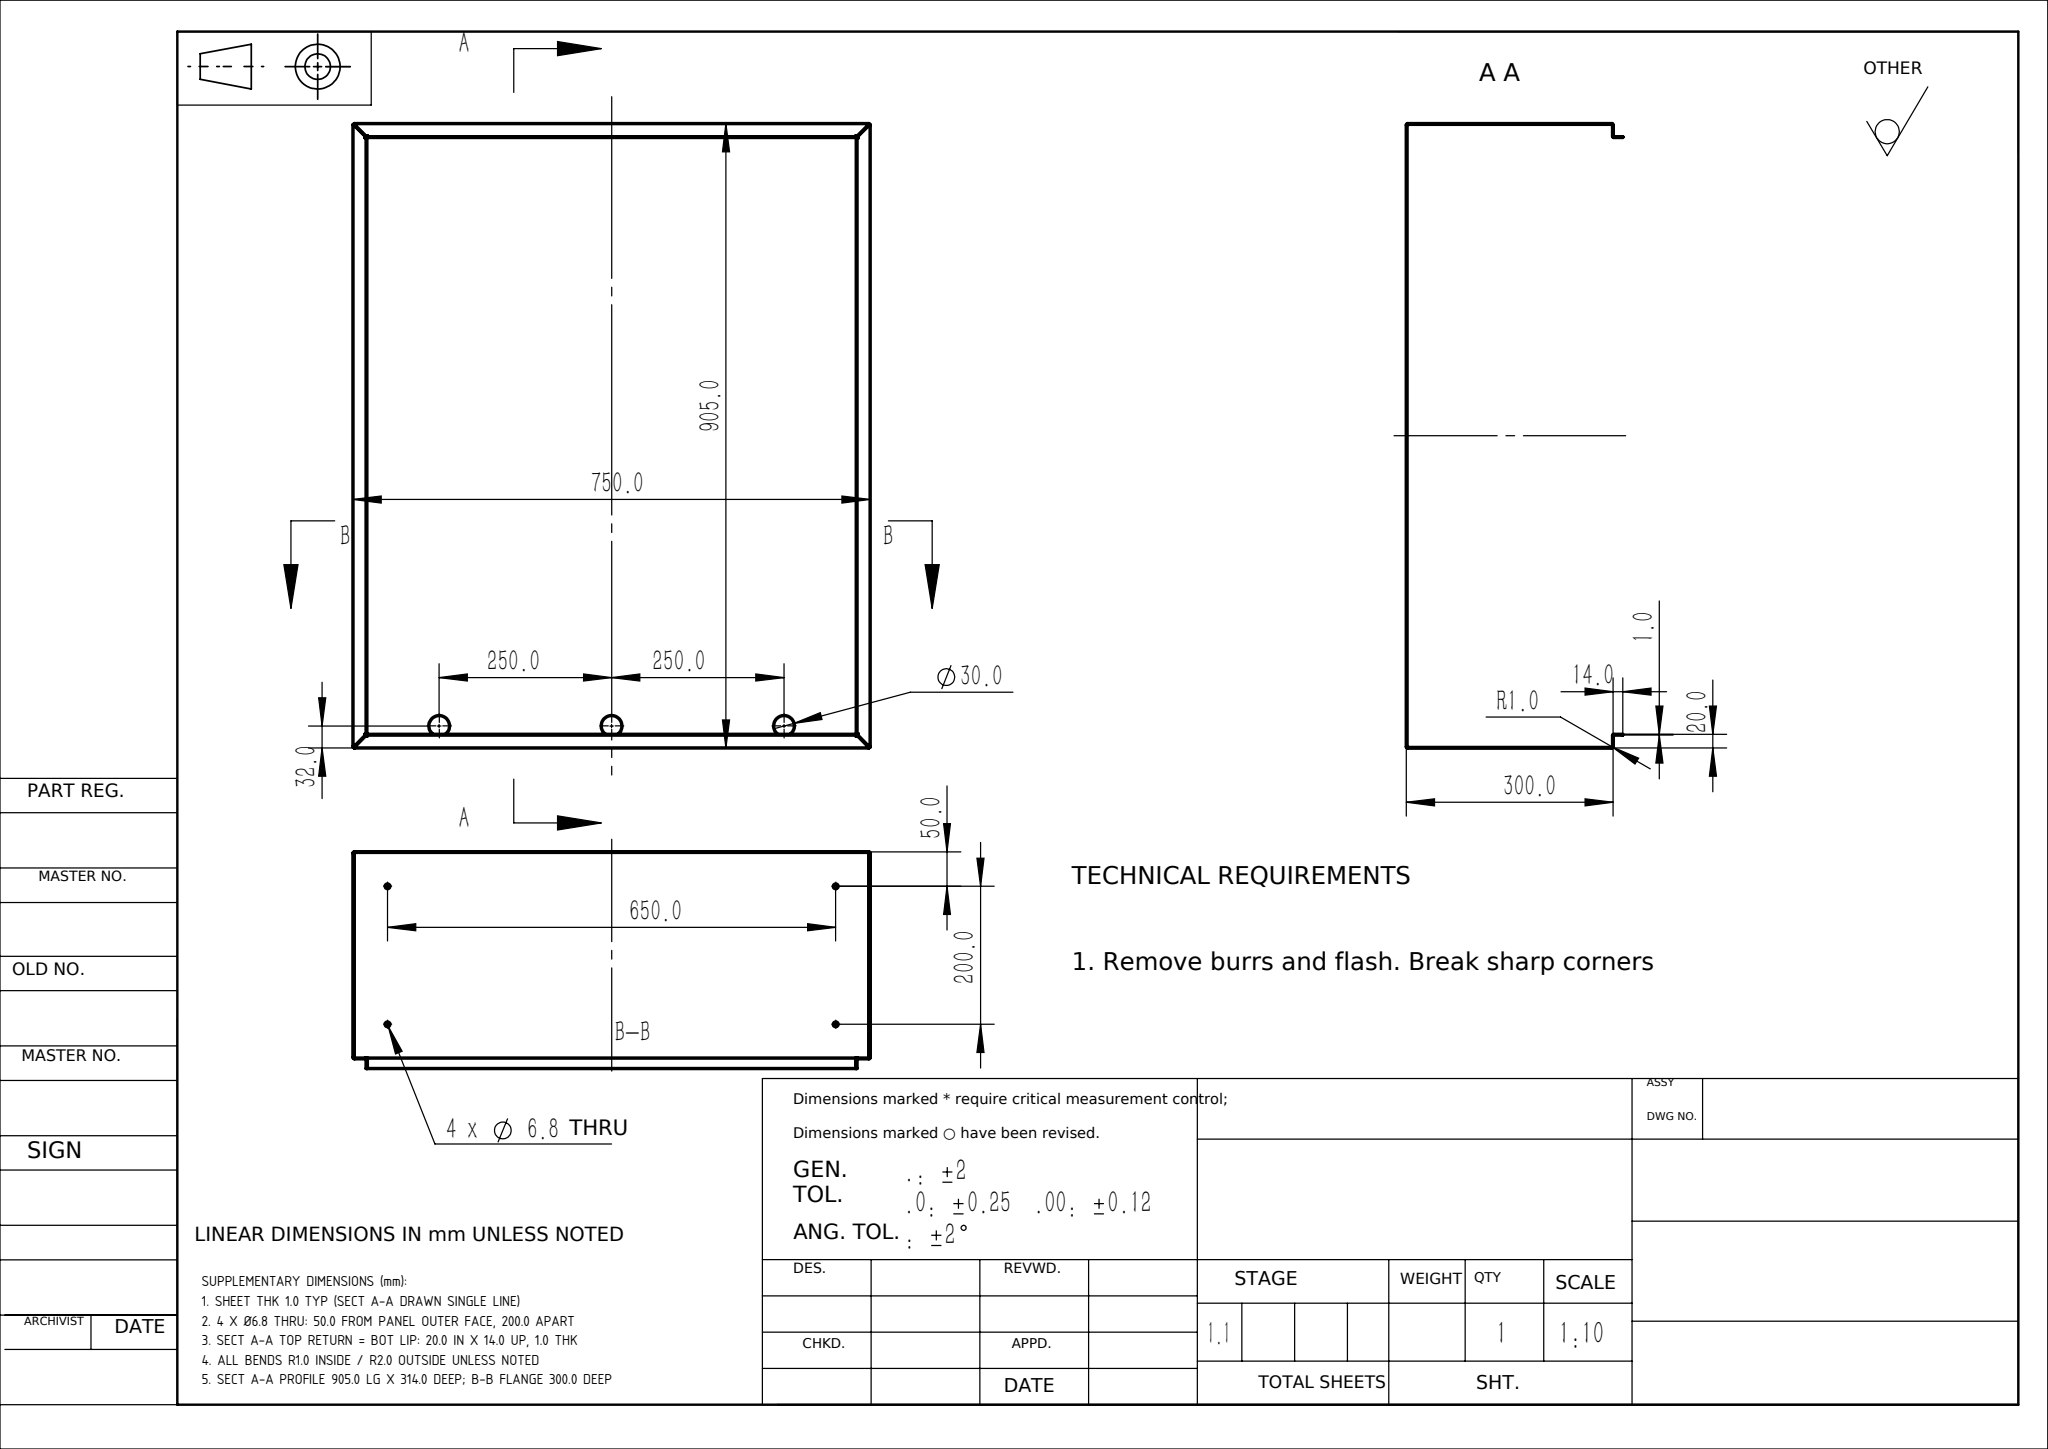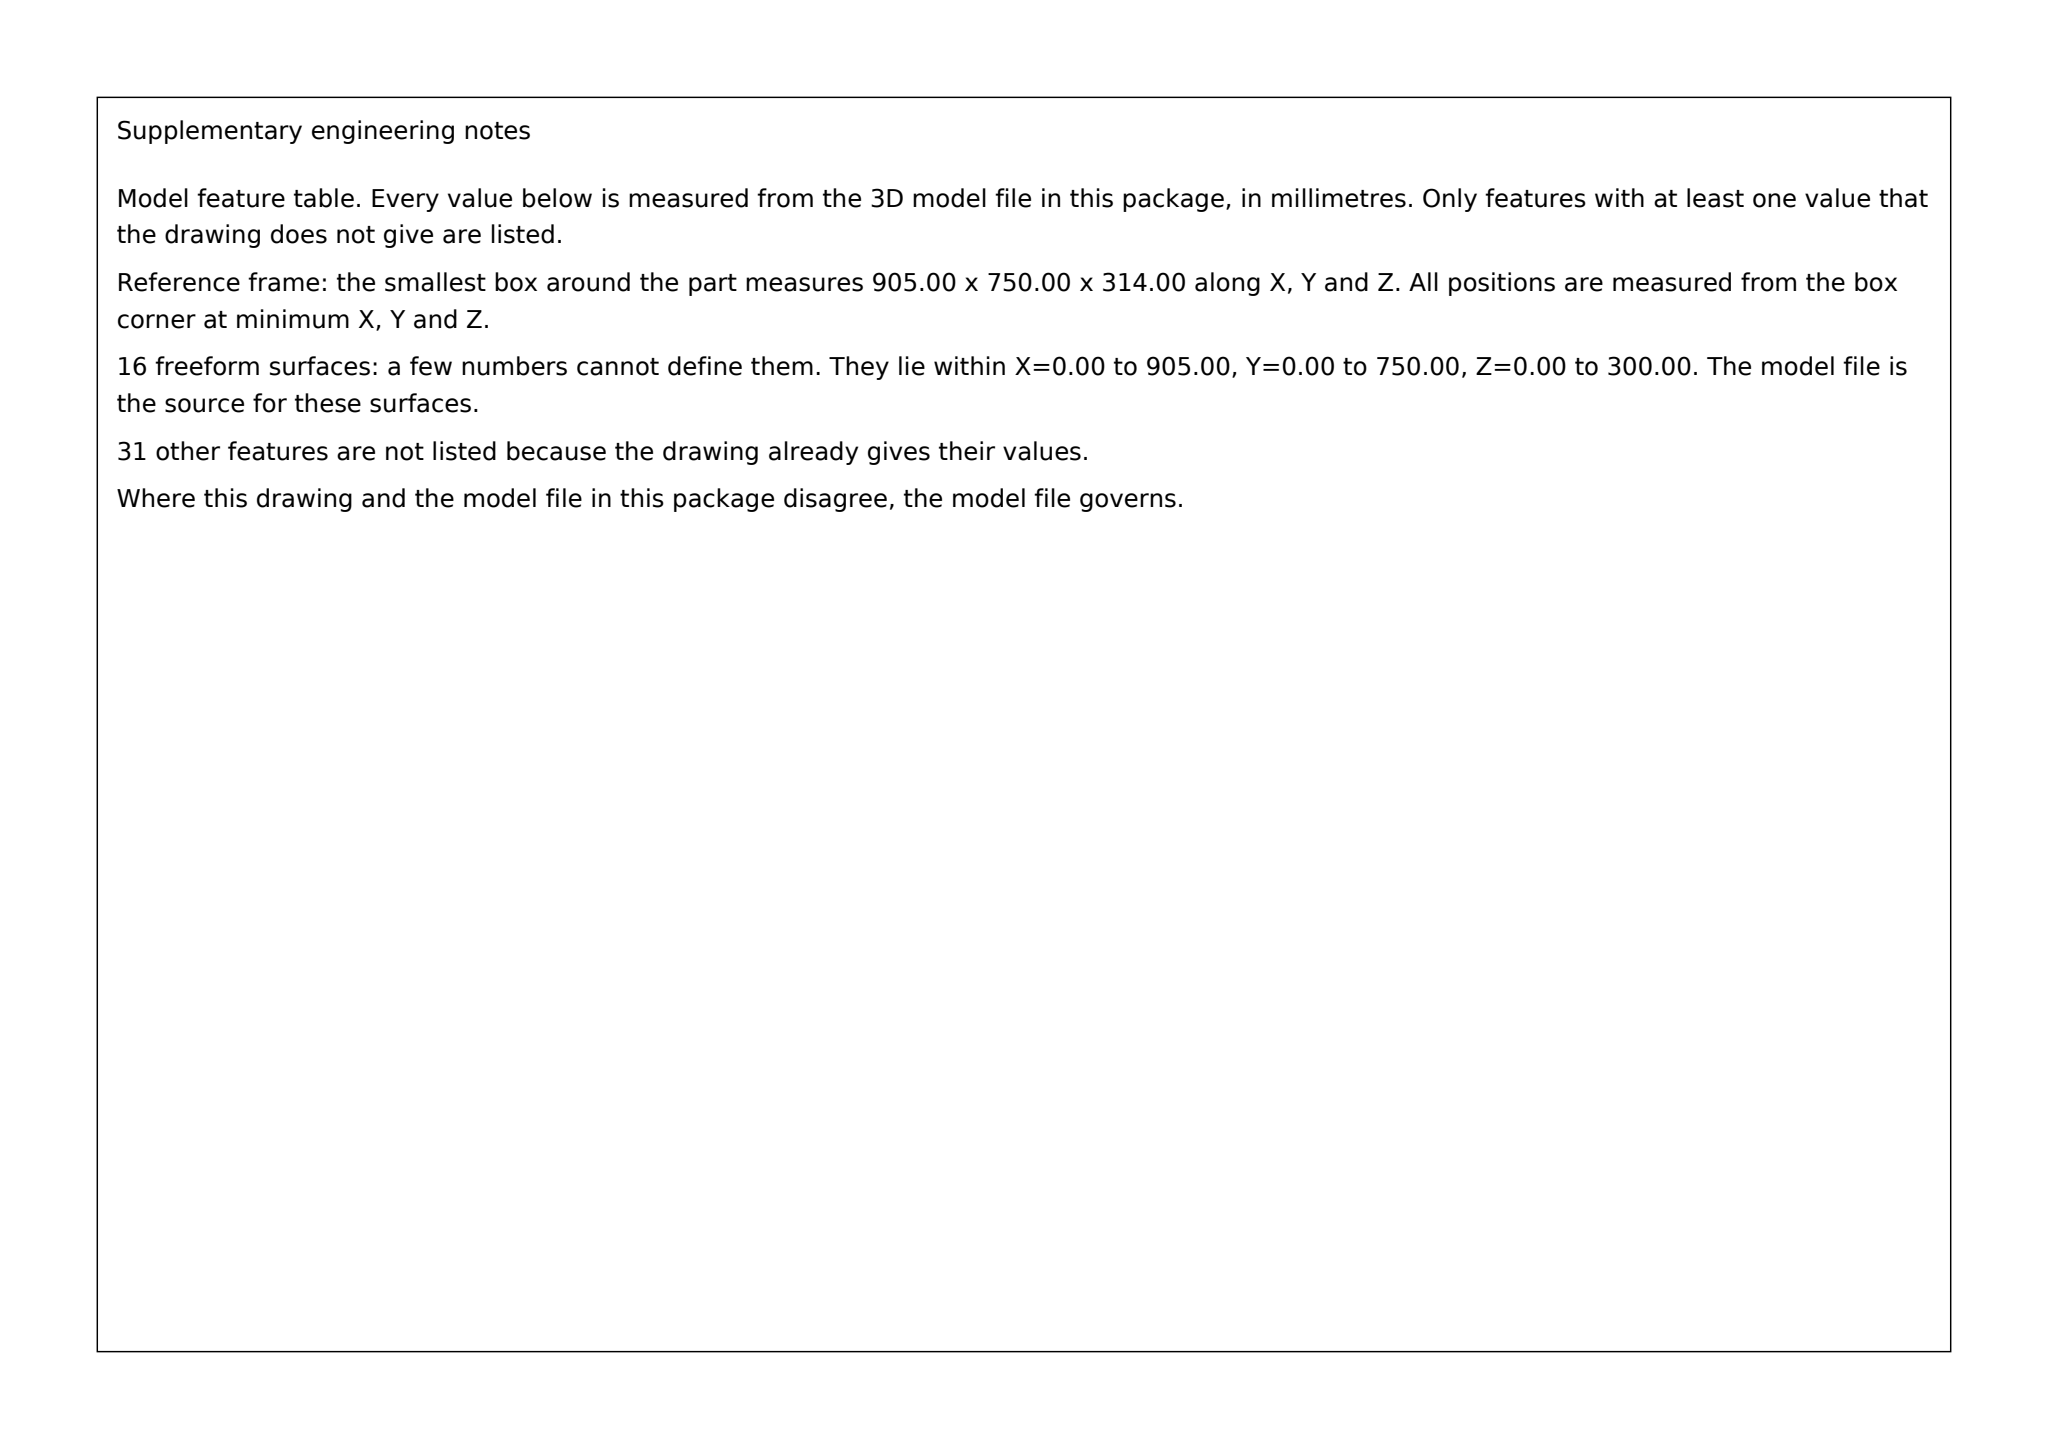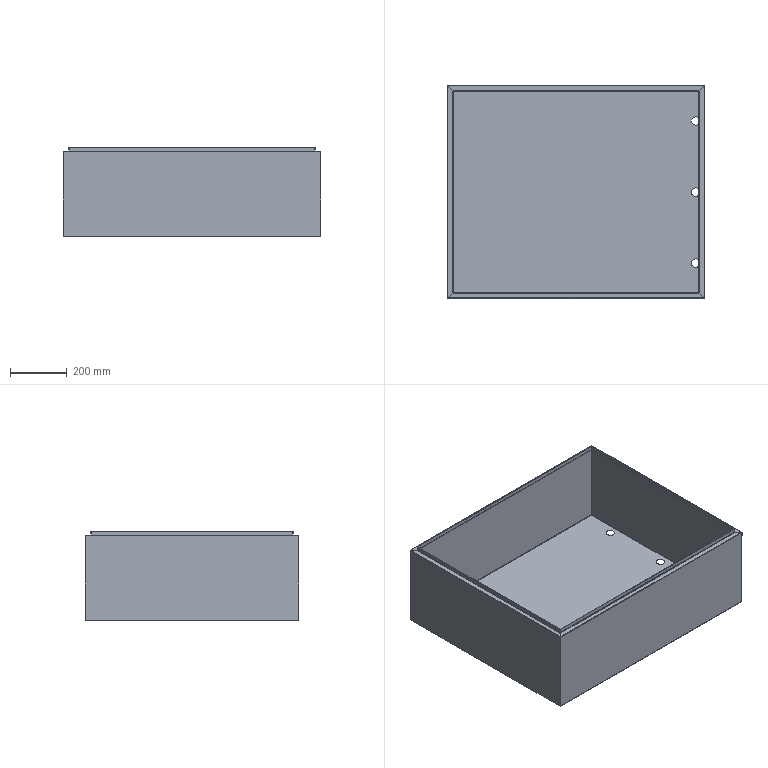Part | SolidWorks | mm | 1 solid | 140 faces | box 905 x 750 x 314 mm | volume 1761002 mm3 | plane 86 | cylinder 38 | spline 16 | commonest cylinder face diameters 4 x12 2 x12 6.8 x8 30 x6